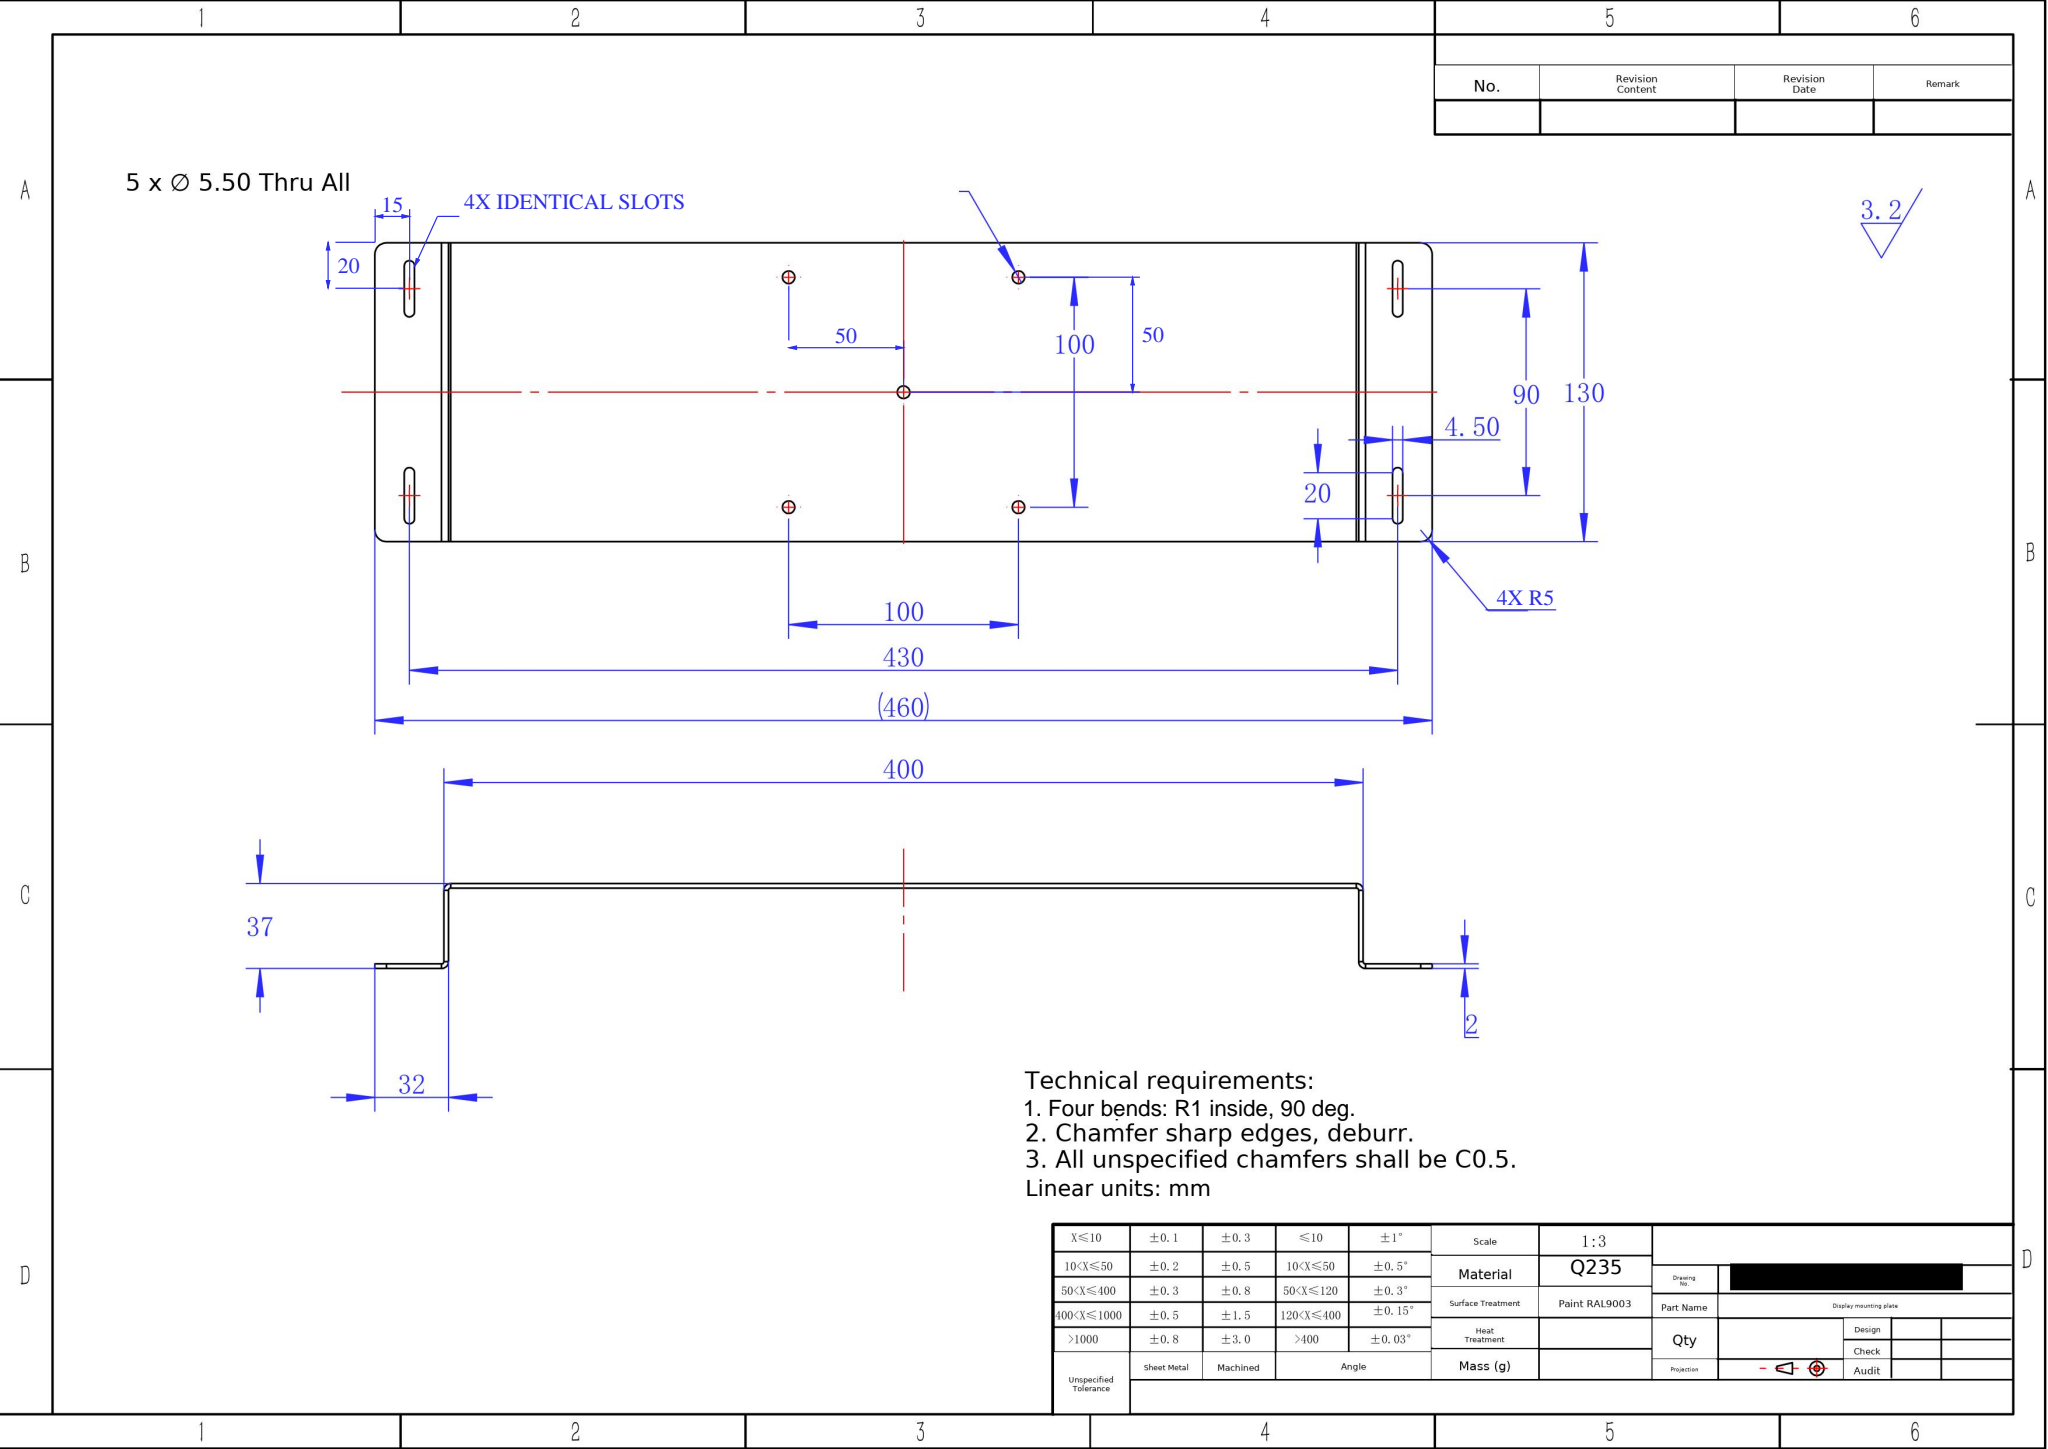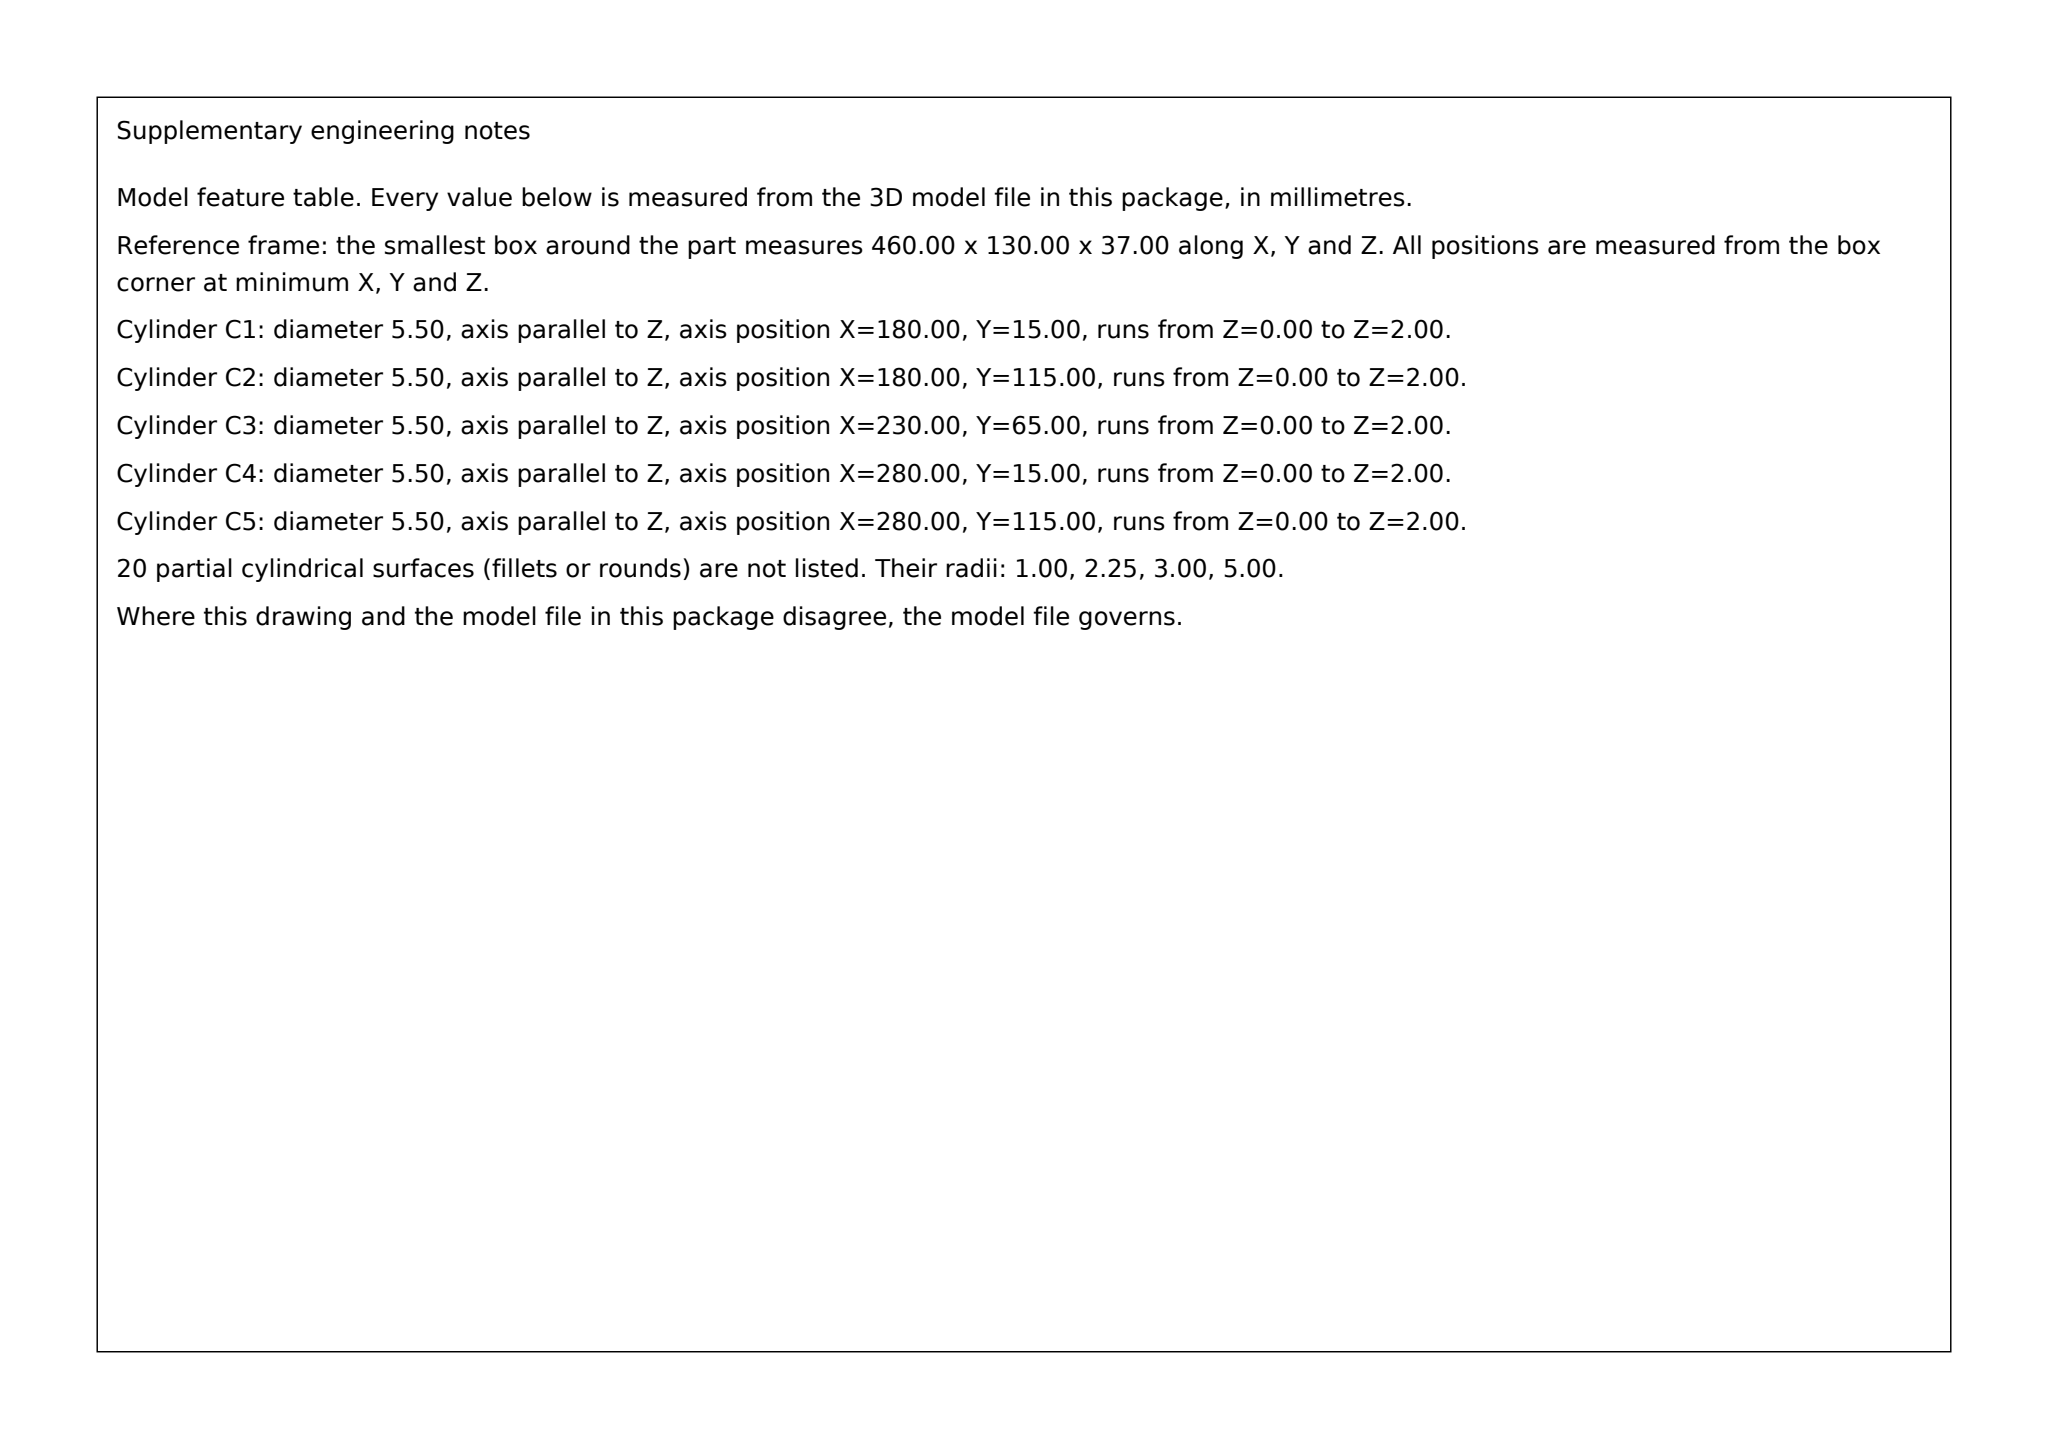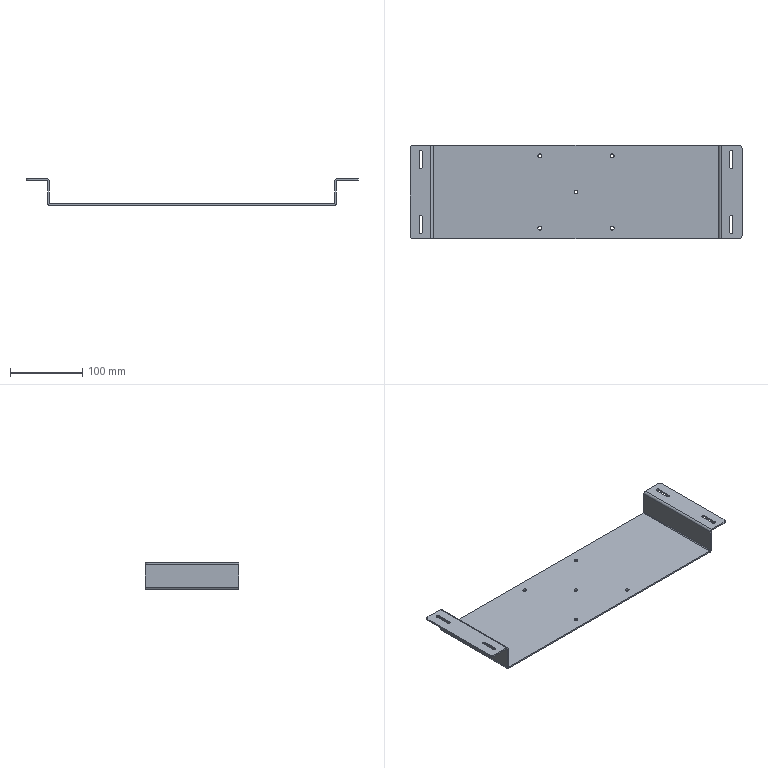Part | SolidWorks | mm | material Q235 | 1 solid | 68 faces | box 460 x 130 x 37 mm | volume 135780 mm3 | plane 38 | cylinder 30 | commonest cylinder face diameters 5.5 x10 4.5 x8 6 x4 2 x4 10 x4